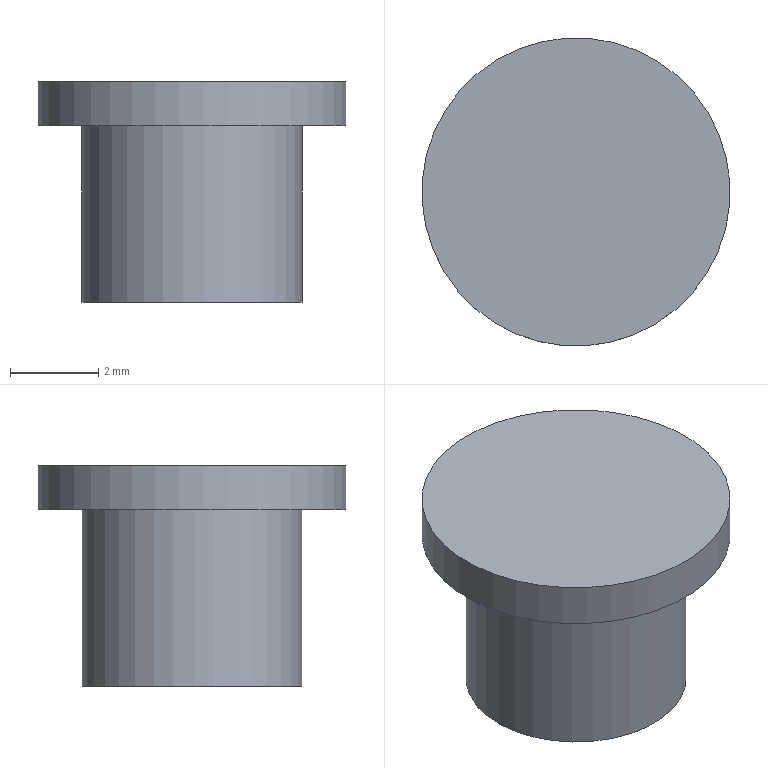Component | NX | CRANK_FIXED_2 | 1 solid | 5 faces | box 7 x 7 x 5 mm | volume 117 mm3 | plane 3 | cylinder 2 | commonest cylinder face diameters 7 x1 5 x1
STEP:
#1=CARTESIAN_POINT('',(0.,0.,0.));
#2=DIRECTION('',(0.,0.,1.));
#3=DIRECTION('',(1.,0.,0.));
#4=AXIS2_PLACEMENT_3D('',#1,#2,#3);
#5=CARTESIAN_POINT('',(-6.869,7.995,-4.49));
#6=VERTEX_POINT('',#5);
#7=CARTESIAN_POINT('',(-10.114,6.685,-4.49));
#8=DIRECTION('',(0.,0.,1.));
#9=DIRECTION('',(0.9273,0.3744,0.));
#10=AXIS2_PLACEMENT_3D('',#7,#8,#9);
#11=CIRCLE('',#10,3.5);
#12=CARTESIAN_POINT('',(-10.114,6.685,-4.49));
#13=DIRECTION('',(0.,0.,1.));
#14=DIRECTION('',(0.9273,0.3744,0.));
#15=AXIS2_PLACEMENT_3D('',#12,#13,#14);
#16=CYLINDRICAL_SURFACE('',#15,3.5);
#17=CARTESIAN_POINT('',(0.,0.));
#18=DIRECTION('',(1.,0.));
#19=VECTOR('',#18,1.);
#20=LINE('',#17,#19);
#21=(GEOMETRIC_REPRESENTATION_CONTEXT(2)PARAMETRIC_REPRESENTATION_CONTEXT()REPRESENTATION_CONTEXT('',''));
#22=DEFINITIONAL_REPRESENTATION('',(#20),#21);
#23=PCURVE('',#16,#22);
#24=CARTESIAN_POINT('',(-10.114,6.685,-4.49));
#25=DIRECTION('',(0.,0.,1.));
#26=DIRECTION('',(0.9273,0.3744,0.));
#27=AXIS2_PLACEMENT_3D('',#24,#25,#26);
#28=PLANE('',#27);
#29=CARTESIAN_POINT('',(0.,0.));
#30=DIRECTION('',(1.,0.));
#31=AXIS2_PLACEMENT_2D('',#29,#30);
#32=CIRCLE('',#31,3.5);
#33=(GEOMETRIC_REPRESENTATION_CONTEXT(2)PARAMETRIC_REPRESENTATION_CONTEXT()REPRESENTATION_CONTEXT('',''));
#34=DEFINITIONAL_REPRESENTATION('',(#32),#33);
#35=PCURVE('',#28,#34);
#36=SURFACE_CURVE('',#11,(#23,#35),.PCURVE_S1.);
#37=EDGE_CURVE('',#6,#6,#36,.T.);
#38=ORIENTED_EDGE('',*,*,#37,.T.);
#39=CARTESIAN_POINT('',(-6.869,7.995,-3.49));
#40=VERTEX_POINT('',#39);
#41=CARTESIAN_POINT('',(-6.869,7.995,-4.49));
#42=CARTESIAN_POINT('',(-6.869,7.995,-3.49));
#43=B_SPLINE_CURVE_WITH_KNOTS('',1,(#41,#42),.UNSPECIFIED.,.F.,.F.,(2,2),(0.,1.),.PIECEWISE_BEZIER_KNOTS.);
#44=CARTESIAN_POINT('',(6.283,0.));
#45=DIRECTION('',(0.,1.));
#46=VECTOR('',#45,1.);
#47=LINE('',#44,#46);
#48=(GEOMETRIC_REPRESENTATION_CONTEXT(2)PARAMETRIC_REPRESENTATION_CONTEXT()REPRESENTATION_CONTEXT('',''));
#49=DEFINITIONAL_REPRESENTATION('',(#47),#48);
#50=PCURVE('',#16,#49);
#51=CARTESIAN_POINT('',(0.,0.));
#52=DIRECTION('',(0.,1.));
#53=VECTOR('',#52,1.);
#54=LINE('',#51,#53);
#55=(GEOMETRIC_REPRESENTATION_CONTEXT(2)PARAMETRIC_REPRESENTATION_CONTEXT()REPRESENTATION_CONTEXT('',''));
#56=DEFINITIONAL_REPRESENTATION('',(#54),#55);
#57=PCURVE('',#16,#56);
#58=SEAM_CURVE('',#43,(#50,#57),.PCURVE_S1.);
#59=EDGE_CURVE('',#6,#40,#58,.T.);
#60=ORIENTED_EDGE('',*,*,#59,.T.);
#61=CARTESIAN_POINT('',(-10.114,6.685,-3.49));
#62=DIRECTION('',(0.,0.,1.));
#63=DIRECTION('',(0.9273,0.3744,0.));
#64=AXIS2_PLACEMENT_3D('',#61,#62,#63);
#65=CIRCLE('',#64,3.5);
#66=CARTESIAN_POINT('',(0.,1.));
#67=DIRECTION('',(1.,0.));
#68=VECTOR('',#67,1.);
#69=LINE('',#66,#68);
#70=(GEOMETRIC_REPRESENTATION_CONTEXT(2)PARAMETRIC_REPRESENTATION_CONTEXT()REPRESENTATION_CONTEXT('',''));
#71=DEFINITIONAL_REPRESENTATION('',(#69),#70);
#72=PCURVE('',#16,#71);
#73=CARTESIAN_POINT('',(-10.114,6.685,-3.49));
#74=DIRECTION('',(0.,0.,1.));
#75=DIRECTION('',(0.9273,0.3744,0.));
#76=AXIS2_PLACEMENT_3D('',#73,#74,#75);
#77=PLANE('',#76);
#78=CARTESIAN_POINT('',(0.,0.));
#79=DIRECTION('',(1.,0.));
#80=AXIS2_PLACEMENT_2D('',#78,#79);
#81=CIRCLE('',#80,3.5);
#82=(GEOMETRIC_REPRESENTATION_CONTEXT(2)PARAMETRIC_REPRESENTATION_CONTEXT()REPRESENTATION_CONTEXT('',''));
#83=DEFINITIONAL_REPRESENTATION('',(#81),#82);
#84=PCURVE('',#77,#83);
#85=SURFACE_CURVE('',#65,(#72,#84),.PCURVE_S1.);
#86=EDGE_CURVE('',#40,#40,#85,.T.);
#87=ORIENTED_EDGE('',*,*,#86,.F.);
#88=ORIENTED_EDGE('',*,*,#59,.F.);
#89=EDGE_LOOP('',(#38,#60,#87,#88));
#90=FACE_BOUND('',#89,.T.);
#91=ADVANCED_FACE('',(#90),#16,.T.);
#92=CARTESIAN_POINT('',(-7.796,7.621,-4.49));
#93=VERTEX_POINT('',#92);
#94=CARTESIAN_POINT('',(-10.114,6.685,-4.49));
#95=DIRECTION('',(0.,0.,-1.));
#96=DIRECTION('',(0.9273,0.3744,0.));
#97=AXIS2_PLACEMENT_3D('',#94,#95,#96);
#98=CIRCLE('',#97,2.5);
#99=CARTESIAN_POINT('',(2.5,0.));
#100=CARTESIAN_POINT('',(2.5,-4.33));
#101=CARTESIAN_POINT('',(-1.25,-2.165));
#102=CARTESIAN_POINT('',(-5.,-0.));
#103=CARTESIAN_POINT('',(-1.25,2.165));
#104=CARTESIAN_POINT('',(2.5,4.33));
#105=CARTESIAN_POINT('',(2.5,0.));
#106=(BOUNDED_CURVE()B_SPLINE_CURVE(2,(#99,#100,#101,#102,#103,#104,#105),.UNSPECIFIED.,.T.,.F.)B_SPLINE_CURVE_WITH_KNOTS((1,2,2,2,2,1),(-2.094,0.,2.094,4.189,6.283,8.378),.UNSPECIFIED.)CURVE()GEOMETRIC_REPRESENTATION_ITEM()RATIONAL_B_SPLINE_CURVE((1.,0.5,1.,0.5,1.,0.5,1.))REPRESENTATION_ITEM(''));
#107=(GEOMETRIC_REPRESENTATION_CONTEXT(2)PARAMETRIC_REPRESENTATION_CONTEXT()REPRESENTATION_CONTEXT('',''));
#108=DEFINITIONAL_REPRESENTATION('',(#106),#107);
#109=PCURVE('',#28,#108);
#110=CARTESIAN_POINT('',(-10.114,6.685,-4.49));
#111=DIRECTION('',(0.,0.,-1.));
#112=DIRECTION('',(-0.9273,-0.3744,0.));
#113=AXIS2_PLACEMENT_3D('',#110,#111,#112);
#114=CYLINDRICAL_SURFACE('',#113,2.5);
#115=CARTESIAN_POINT('',(3.142,0.));
#116=DIRECTION('',(1.,0.));
#117=VECTOR('',#116,1.);
#118=LINE('',#115,#117);
#119=(GEOMETRIC_REPRESENTATION_CONTEXT(2)PARAMETRIC_REPRESENTATION_CONTEXT()REPRESENTATION_CONTEXT('',''));
#120=DEFINITIONAL_REPRESENTATION('',(#118),#119);
#121=PCURVE('',#114,#120);
#122=SURFACE_CURVE('',#98,(#109,#121),.PCURVE_S1.);
#123=EDGE_CURVE('',#93,#93,#122,.T.);
#124=ORIENTED_EDGE('',*,*,#123,.F.);
#125=EDGE_LOOP('',(#124));
#126=FACE_BOUND('',#125,.T.);
#127=ORIENTED_EDGE('',*,*,#37,.F.);
#128=EDGE_LOOP('',(#127));
#129=FACE_BOUND('',#128,.T.);
#130=ADVANCED_FACE('',(#126,#129),#28,.F.);
#131=ORIENTED_EDGE('',*,*,#86,.T.);
#132=EDGE_LOOP('',(#131));
#133=FACE_BOUND('',#132,.T.);
#134=ADVANCED_FACE('',(#133),#77,.T.);
#135=ORIENTED_EDGE('',*,*,#123,.T.);
#136=CARTESIAN_POINT('',(-7.796,7.621,-8.49));
#137=VERTEX_POINT('',#136);
#138=CARTESIAN_POINT('',(-7.796,7.621,-4.49));
#139=CARTESIAN_POINT('',(-7.796,7.621,-8.49));
#140=B_SPLINE_CURVE_WITH_KNOTS('',1,(#138,#139),.UNSPECIFIED.,.F.,.F.,(2,2),(0.,4.),.PIECEWISE_BEZIER_KNOTS.);
#141=CARTESIAN_POINT('',(9.425,0.));
#142=DIRECTION('',(0.,1.));
#143=VECTOR('',#142,1.);
#144=LINE('',#141,#143);
#145=(GEOMETRIC_REPRESENTATION_CONTEXT(2)PARAMETRIC_REPRESENTATION_CONTEXT()REPRESENTATION_CONTEXT('',''));
#146=DEFINITIONAL_REPRESENTATION('',(#144),#145);
#147=PCURVE('',#114,#146);
#148=CARTESIAN_POINT('',(3.142,0.));
#149=DIRECTION('',(0.,1.));
#150=VECTOR('',#149,1.);
#151=LINE('',#148,#150);
#152=(GEOMETRIC_REPRESENTATION_CONTEXT(2)PARAMETRIC_REPRESENTATION_CONTEXT()REPRESENTATION_CONTEXT('',''));
#153=DEFINITIONAL_REPRESENTATION('',(#151),#152);
#154=PCURVE('',#114,#153);
#155=SEAM_CURVE('',#140,(#147,#154),.PCURVE_S1.);
#156=EDGE_CURVE('',#93,#137,#155,.T.);
#157=ORIENTED_EDGE('',*,*,#156,.T.);
#158=CARTESIAN_POINT('',(-10.114,6.685,-8.49));
#159=DIRECTION('',(0.,0.,-1.));
#160=DIRECTION('',(0.9273,0.3744,0.));
#161=AXIS2_PLACEMENT_3D('',#158,#159,#160);
#162=CIRCLE('',#161,2.5);
#163=CARTESIAN_POINT('',(3.142,4.));
#164=DIRECTION('',(1.,0.));
#165=VECTOR('',#164,1.);
#166=LINE('',#163,#165);
#167=(GEOMETRIC_REPRESENTATION_CONTEXT(2)PARAMETRIC_REPRESENTATION_CONTEXT()REPRESENTATION_CONTEXT('',''));
#168=DEFINITIONAL_REPRESENTATION('',(#166),#167);
#169=PCURVE('',#114,#168);
#170=CARTESIAN_POINT('',(-10.114,6.685,-8.49));
#171=DIRECTION('',(0.,0.,-1.));
#172=DIRECTION('',(-0.9273,-0.3744,0.));
#173=AXIS2_PLACEMENT_3D('',#170,#171,#172);
#174=PLANE('',#173);
#175=CARTESIAN_POINT('',(0.,0.));
#176=DIRECTION('',(-1.,0.));
#177=AXIS2_PLACEMENT_2D('',#175,#176);
#178=CIRCLE('',#177,2.5);
#179=(GEOMETRIC_REPRESENTATION_CONTEXT(2)PARAMETRIC_REPRESENTATION_CONTEXT()REPRESENTATION_CONTEXT('',''));
#180=DEFINITIONAL_REPRESENTATION('',(#178),#179);
#181=PCURVE('',#174,#180);
#182=SURFACE_CURVE('',#162,(#169,#181),.PCURVE_S1.);
#183=EDGE_CURVE('',#137,#137,#182,.T.);
#184=ORIENTED_EDGE('',*,*,#183,.F.);
#185=ORIENTED_EDGE('',*,*,#156,.F.);
#186=EDGE_LOOP('',(#135,#157,#184,#185));
#187=FACE_BOUND('',#186,.T.);
#188=ADVANCED_FACE('',(#187),#114,.T.);
#189=ORIENTED_EDGE('',*,*,#183,.T.);
#190=EDGE_LOOP('',(#189));
#191=FACE_BOUND('',#190,.T.);
#192=ADVANCED_FACE('',(#191),#174,.T.);
#193=CLOSED_SHELL('',(#91,#130,#134,#188,#192));
#194=MANIFOLD_SOLID_BREP('',#193);
#195=(LENGTH_UNIT()NAMED_UNIT(*)SI_UNIT(.MILLI.,.METRE.));
#196=UNCERTAINTY_MEASURE_WITH_UNIT(LENGTH_MEASURE(0.00001),#195,'','');
#197=(NAMED_UNIT(*)PLANE_ANGLE_UNIT()SI_UNIT($,.RADIAN.));
#198=(NAMED_UNIT(*)SI_UNIT($,.STERADIAN.)SOLID_ANGLE_UNIT());
#199=(GEOMETRIC_REPRESENTATION_CONTEXT(3)GLOBAL_UNCERTAINTY_ASSIGNED_CONTEXT((#196))GLOBAL_UNIT_ASSIGNED_CONTEXT((#195,#197,#198))REPRESENTATION_CONTEXT('',''));
#200=ADVANCED_BREP_SHAPE_REPRESENTATION('',(#4,#194),#199);